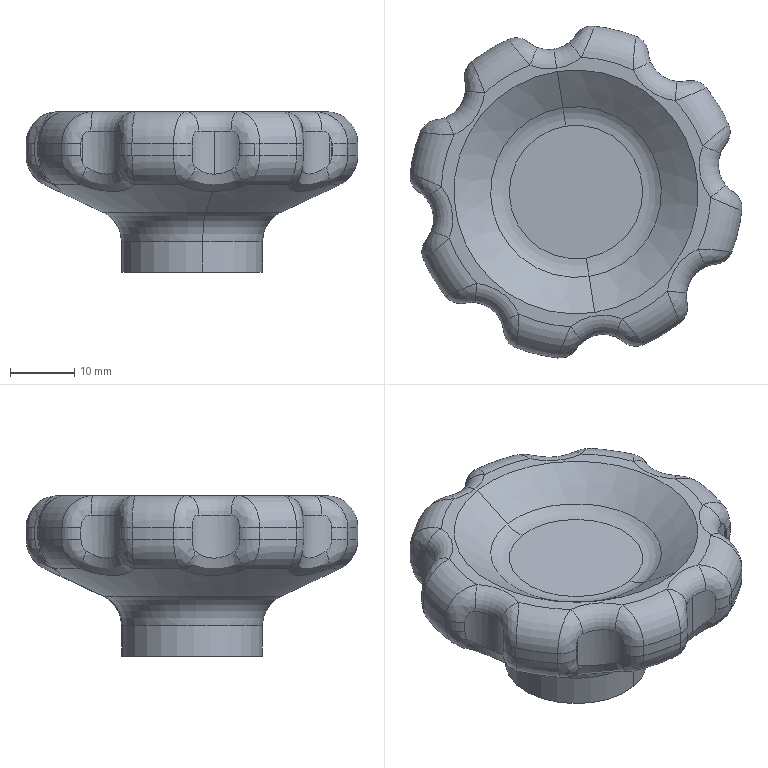Component | SolidWorks | KnurledWheel.1-1 | 1 solid | 120 faces | volume 25004 mm3 | cylinder 43 | spline 40 | torus 29 | cone 4 | plane 4 | commonest cylinder face diameters 6 x20 10 x11 52 x8 8 x2 22 x2